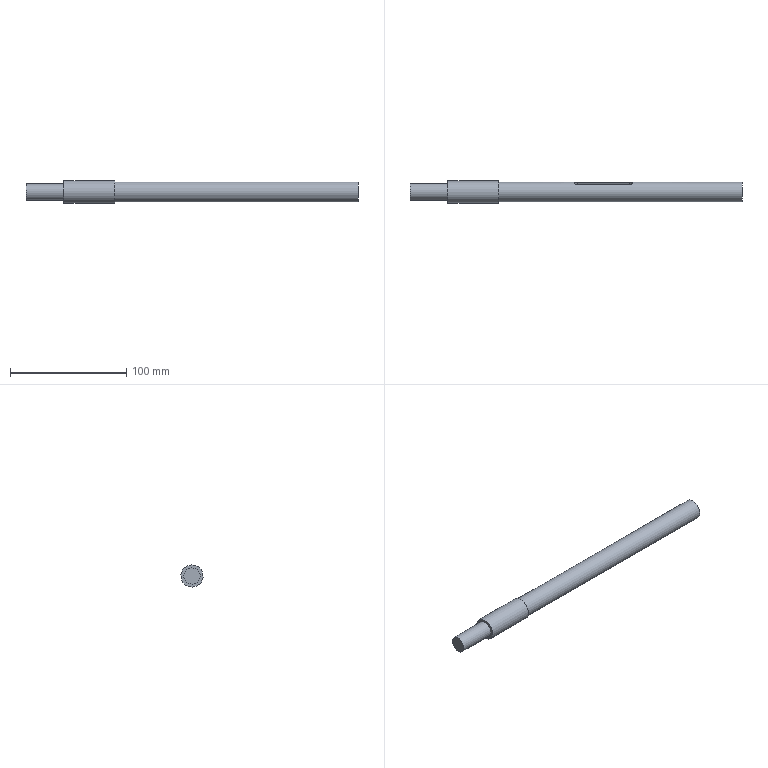Component | NX | SHAFT | 1 solid | 12 faces | box 285 x 19 x 19 mm | volume 64194 mm3 | plane 7 | cylinder 5 | commonest cylinder face diameters 5 x2 17 x1 14 x1 19 x1
STEP:
#1=CARTESIAN_POINT('',(0.,0.,0.));
#2=DIRECTION('',(0.,0.,1.));
#3=DIRECTION('',(1.,0.,0.));
#4=AXIS2_PLACEMENT_3D('',#1,#2,#3);
#5=CARTESIAN_POINT('',(190.,-3.867,130.57));
#6=VERTEX_POINT('',#5);
#7=CARTESIAN_POINT('',(190.,-0.,123.));
#8=DIRECTION('',(1.,0.,0.));
#9=DIRECTION('',(0.,-0.4549,0.8906));
#10=AXIS2_PLACEMENT_3D('',#7,#8,#9);
#11=CIRCLE('',#10,8.5);
#12=CARTESIAN_POINT('',(-19.,-0.,123.));
#13=DIRECTION('',(1.,0.,0.));
#14=DIRECTION('',(0.,-0.4549,0.8906));
#15=AXIS2_PLACEMENT_3D('',#12,#13,#14);
#16=CYLINDRICAL_SURFACE('',#15,8.5);
#17=CARTESIAN_POINT('',(0.,209.));
#18=DIRECTION('',(1.,0.));
#19=VECTOR('',#18,1.);
#20=LINE('',#17,#19);
#21=(GEOMETRIC_REPRESENTATION_CONTEXT(2)PARAMETRIC_REPRESENTATION_CONTEXT()REPRESENTATION_CONTEXT('',''));
#22=DEFINITIONAL_REPRESENTATION('',(#20),#21);
#23=PCURVE('',#16,#22);
#24=CARTESIAN_POINT('',(190.,-0.,123.));
#25=DIRECTION('',(1.,0.,0.));
#26=DIRECTION('',(0.,-0.4549,0.8906));
#27=AXIS2_PLACEMENT_3D('',#24,#25,#26);
#28=PLANE('',#27);
#29=CARTESIAN_POINT('',(0.,0.));
#30=DIRECTION('',(1.,-0.));
#31=AXIS2_PLACEMENT_2D('',#29,#30);
#32=CIRCLE('',#31,8.5);
#33=(GEOMETRIC_REPRESENTATION_CONTEXT(2)PARAMETRIC_REPRESENTATION_CONTEXT()REPRESENTATION_CONTEXT('',''));
#34=DEFINITIONAL_REPRESENTATION('',(#32),#33);
#35=PCURVE('',#28,#34);
#36=SURFACE_CURVE('',#11,(#23,#35),.PCURVE_S1.);
#37=EDGE_CURVE('',#6,#6,#36,.T.);
#38=ORIENTED_EDGE('',*,*,#37,.F.);
#39=CARTESIAN_POINT('',(-19.,-3.867,130.57));
#40=VERTEX_POINT('',#39);
#41=CARTESIAN_POINT('',(-19.,-3.867,130.57));
#42=CARTESIAN_POINT('',(190.,-3.867,130.57));
#43=B_SPLINE_CURVE_WITH_KNOTS('',1,(#41,#42),.UNSPECIFIED.,.F.,.F.,(2,2),(0.,209.),.PIECEWISE_BEZIER_KNOTS.);
#44=CARTESIAN_POINT('',(0.,0.));
#45=DIRECTION('',(0.,1.));
#46=VECTOR('',#45,1.);
#47=LINE('',#44,#46);
#48=(GEOMETRIC_REPRESENTATION_CONTEXT(2)PARAMETRIC_REPRESENTATION_CONTEXT()REPRESENTATION_CONTEXT('',''));
#49=DEFINITIONAL_REPRESENTATION('',(#47),#48);
#50=PCURVE('',#16,#49);
#51=CARTESIAN_POINT('',(6.283,0.));
#52=DIRECTION('',(0.,1.));
#53=VECTOR('',#52,1.);
#54=LINE('',#51,#53);
#55=(GEOMETRIC_REPRESENTATION_CONTEXT(2)PARAMETRIC_REPRESENTATION_CONTEXT()REPRESENTATION_CONTEXT('',''));
#56=DEFINITIONAL_REPRESENTATION('',(#54),#55);
#57=PCURVE('',#16,#56);
#58=SEAM_CURVE('',#43,(#50,#57),.PCURVE_S1.);
#59=EDGE_CURVE('',#40,#6,#58,.T.);
#60=ORIENTED_EDGE('',*,*,#59,.F.);
#61=CARTESIAN_POINT('',(-19.,-0.,123.));
#62=DIRECTION('',(1.,0.,0.));
#63=DIRECTION('',(0.,-0.4549,0.8906));
#64=AXIS2_PLACEMENT_3D('',#61,#62,#63);
#65=CIRCLE('',#64,8.5);
#66=CARTESIAN_POINT('',(0.,0.));
#67=DIRECTION('',(1.,0.));
#68=VECTOR('',#67,1.);
#69=LINE('',#66,#68);
#70=(GEOMETRIC_REPRESENTATION_CONTEXT(2)PARAMETRIC_REPRESENTATION_CONTEXT()REPRESENTATION_CONTEXT('',''));
#71=DEFINITIONAL_REPRESENTATION('',(#69),#70);
#72=PCURVE('',#16,#71);
#73=CARTESIAN_POINT('',(-19.,-0.,123.));
#74=DIRECTION('',(1.,0.,0.));
#75=DIRECTION('',(0.,-0.4549,0.8906));
#76=AXIS2_PLACEMENT_3D('',#73,#74,#75);
#77=PLANE('',#76);
#78=CARTESIAN_POINT('',(-0.,-0.));
#79=DIRECTION('',(1.,-0.));
#80=AXIS2_PLACEMENT_2D('',#78,#79);
#81=CIRCLE('',#80,8.5);
#82=(GEOMETRIC_REPRESENTATION_CONTEXT(2)PARAMETRIC_REPRESENTATION_CONTEXT()REPRESENTATION_CONTEXT('',''));
#83=DEFINITIONAL_REPRESENTATION('',(#81),#82);
#84=PCURVE('',#77,#83);
#85=SURFACE_CURVE('',#65,(#72,#84),.PCURVE_S1.);
#86=EDGE_CURVE('',#40,#40,#85,.T.);
#87=ORIENTED_EDGE('',*,*,#86,.T.);
#88=ORIENTED_EDGE('',*,*,#59,.T.);
#89=EDGE_LOOP('',(#38,#60,#87,#88));
#90=FACE_BOUND('',#89,.T.);
#91=CARTESIAN_POINT('',(48.5,6.098,128.922));
#92=VERTEX_POINT('',#91);
#93=CARTESIAN_POINT('',(48.5,8.372,124.469));
#94=VERTEX_POINT('',#93);
#95=CARTESIAN_POINT('',(48.5,6.098,128.922));
#96=CARTESIAN_POINT('',(48.227,6.098,128.922));
#97=CARTESIAN_POINT('',(47.95,6.132,128.887));
#98=CARTESIAN_POINT('',(47.693,6.194,128.821));
#99=CARTESIAN_POINT('',(47.436,6.257,128.754));
#100=CARTESIAN_POINT('',(47.191,6.349,128.654));
#101=CARTESIAN_POINT('',(46.977,6.459,128.526));
#102=CARTESIAN_POINT('',(46.757,6.572,128.394));
#103=CARTESIAN_POINT('',(46.564,6.706,128.228));
#104=CARTESIAN_POINT('',(46.411,6.845,128.039));
#105=CARTESIAN_POINT('',(46.256,6.987,127.846));
#106=CARTESIAN_POINT('',(46.139,7.139,127.622));
#107=CARTESIAN_POINT('',(46.071,7.282,127.385));
#108=CARTESIAN_POINT('',(46.006,7.421,127.153));
#109=CARTESIAN_POINT('',(45.985,7.556,126.902));
#110=CARTESIAN_POINT('',(46.011,7.675,126.653));
#111=CARTESIAN_POINT('',(46.037,7.79,126.411));
#112=CARTESIAN_POINT('',(46.108,7.893,126.163));
#113=CARTESIAN_POINT('',(46.217,7.978,125.932));
#114=CARTESIAN_POINT('',(46.327,8.064,125.698));
#115=CARTESIAN_POINT('',(46.479,8.134,125.475));
#116=CARTESIAN_POINT('',(46.662,8.189,125.28));
#117=CARTESIAN_POINT('',(46.851,8.245,125.078));
#118=CARTESIAN_POINT('',(47.078,8.286,124.902));
#119=CARTESIAN_POINT('',(47.326,8.314,124.768));
#120=CARTESIAN_POINT('',(47.575,8.343,124.634));
#121=CARTESIAN_POINT('',(47.853,8.36,124.54));
#122=CARTESIAN_POINT('',(48.135,8.367,124.497));
#123=CARTESIAN_POINT('',(48.255,8.37,124.478));
#124=CARTESIAN_POINT('',(48.378,8.372,124.469));
#125=CARTESIAN_POINT('',(48.5,8.372,124.469));
#126=B_SPLINE_CURVE_WITH_KNOTS('',3,(#95,#96,#97,#98,#99,#100,#101,#102,#103,#104,#105,#106,#107,#108,#109,#110,#111,#112,#113,#114,#115,#116,#117,#118,#119,#120,#121,#122,#123,#124,#125),.UNSPECIFIED.,.F.,.F.,(4,3,3,3,3,3,3,3,3,3,4),(0.,0.1042,0.2083,0.3152,0.4244,0.5305,0.6332,0.7372,0.845,0.9539,1.),.UNSPECIFIED.);
#127=CARTESIAN_POINT('',(5.011,67.5));
#128=CARTESIAN_POINT('',(5.011,67.44));
#129=CARTESIAN_POINT('',(5.01,67.321));
#130=CARTESIAN_POINT('',(5.008,67.142));
#131=CARTESIAN_POINT('',(5.004,66.965));
#132=CARTESIAN_POINT('',(4.999,66.792));
#133=CARTESIAN_POINT('',(4.992,66.623));
#134=CARTESIAN_POINT('',(4.983,66.458));
#135=CARTESIAN_POINT('',(4.974,66.298));
#136=CARTESIAN_POINT('',(4.962,66.145));
#137=CARTESIAN_POINT('',(4.95,65.999));
#138=CARTESIAN_POINT('',(4.937,65.862));
#139=CARTESIAN_POINT('',(4.922,65.731));
#140=CARTESIAN_POINT('',(4.906,65.61));
#141=CARTESIAN_POINT('',(4.89,65.498));
#142=CARTESIAN_POINT('',(4.873,65.397));
#143=CARTESIAN_POINT('',(4.854,65.306));
#144=CARTESIAN_POINT('',(4.835,65.226));
#145=CARTESIAN_POINT('',(4.816,65.157));
#146=CARTESIAN_POINT('',(4.796,65.1));
#147=CARTESIAN_POINT('',(4.776,65.056));
#148=CARTESIAN_POINT('',(4.755,65.024));
#149=CARTESIAN_POINT('',(4.734,65.005));
#150=CARTESIAN_POINT('',(4.713,64.998));
#151=CARTESIAN_POINT('',(4.691,65.004));
#152=CARTESIAN_POINT('',(4.671,65.023));
#153=CARTESIAN_POINT('',(4.65,65.055));
#154=CARTESIAN_POINT('',(4.629,65.1));
#155=CARTESIAN_POINT('',(4.609,65.157));
#156=CARTESIAN_POINT('',(4.59,65.225));
#157=CARTESIAN_POINT('',(4.571,65.305));
#158=CARTESIAN_POINT('',(4.552,65.396));
#159=CARTESIAN_POINT('',(4.535,65.498));
#160=CARTESIAN_POINT('',(4.518,65.609));
#161=CARTESIAN_POINT('',(4.503,65.729));
#162=CARTESIAN_POINT('',(4.488,65.859));
#163=CARTESIAN_POINT('',(4.475,65.998));
#164=CARTESIAN_POINT('',(4.462,66.144));
#165=CARTESIAN_POINT('',(4.451,66.297));
#166=CARTESIAN_POINT('',(4.442,66.455));
#167=CARTESIAN_POINT('',(4.433,66.62));
#168=CARTESIAN_POINT('',(4.426,66.79));
#169=CARTESIAN_POINT('',(4.421,66.964));
#170=CARTESIAN_POINT('',(4.417,67.139));
#171=CARTESIAN_POINT('',(4.414,67.319));
#172=CARTESIAN_POINT('',(4.414,67.44));
#173=CARTESIAN_POINT('',(4.414,67.5));
#174=B_SPLINE_CURVE_WITH_KNOTS('',3,(#127,#128,#129,#130,#131,#132,#133,#134,#135,#136,#137,#138,#139,#140,#141,#142,#143,#144,#145,#146,#147,#148,#149,#150,#151,#152,#153,#154,#155,#156,#157,#158,#159,#160,#161,#162,#163,#164,#165,#166,#167,#168,#169,#170,#171,#172,#173),.UNSPECIFIED.,.F.,.F.,(4,1,1,1,1,1,1,1,1,1,1,1,1,1,1,1,1,1,1,1,1,1,1,1,1,1,1,1,1,1,1,1,1,1,1,1,1,1,1,1,1,1,1,1,4),(0.,0.02273,0.04545,0.06818,0.09091,0.1136,0.1364,0.1591,0.1818,0.2045,0.2273,0.25,0.2727,0.2955,0.3182,0.3409,0.3636,0.3864,0.4091,0.4318,0.4545,0.4773,0.5,0.5227,0.5455,0.5682,0.5909,0.6136,0.6364,0.6591,0.6818,0.7045,0.7273,0.75,0.7727,0.7955,0.8182,0.8409,0.8636,0.8864,0.9091,0.9318,0.9545,0.9773,1.),.QUASI_UNIFORM_KNOTS.);
#175=(GEOMETRIC_REPRESENTATION_CONTEXT(2)PARAMETRIC_REPRESENTATION_CONTEXT()REPRESENTATION_CONTEXT('',''));
#176=DEFINITIONAL_REPRESENTATION('',(#174),#175);
#177=PCURVE('',#16,#176);
#178=CARTESIAN_POINT('',(48.5,44.528,145.744));
#179=DIRECTION('',(0.,-0.8906,-0.4549));
#180=DIRECTION('',(1.,0.,0.));
#181=AXIS2_PLACEMENT_3D('',#178,#179,#180);
#182=CYLINDRICAL_SURFACE('',#181,2.5);
#183=CARTESIAN_POINT('',(1.571,41.876));
#184=CARTESIAN_POINT('',(1.595,41.876));
#185=CARTESIAN_POINT('',(1.642,41.875));
#186=CARTESIAN_POINT('',(1.714,41.869));
#187=CARTESIAN_POINT('',(1.786,41.859));
#188=CARTESIAN_POINT('',(1.858,41.846));
#189=CARTESIAN_POINT('',(1.929,41.829));
#190=CARTESIAN_POINT('',(2.,41.81));
#191=CARTESIAN_POINT('',(2.072,41.788));
#192=CARTESIAN_POINT('',(2.143,41.764));
#193=CARTESIAN_POINT('',(2.214,41.739));
#194=CARTESIAN_POINT('',(2.285,41.713));
#195=CARTESIAN_POINT('',(2.356,41.686));
#196=CARTESIAN_POINT('',(2.427,41.659));
#197=CARTESIAN_POINT('',(2.498,41.633));
#198=CARTESIAN_POINT('',(2.569,41.608));
#199=CARTESIAN_POINT('',(2.64,41.585));
#200=CARTESIAN_POINT('',(2.711,41.564));
#201=CARTESIAN_POINT('',(2.783,41.545));
#202=CARTESIAN_POINT('',(2.854,41.529));
#203=CARTESIAN_POINT('',(2.926,41.516));
#204=CARTESIAN_POINT('',(2.997,41.507));
#205=CARTESIAN_POINT('',(3.069,41.501));
#206=CARTESIAN_POINT('',(3.141,41.499));
#207=CARTESIAN_POINT('',(3.213,41.501));
#208=CARTESIAN_POINT('',(3.284,41.507));
#209=CARTESIAN_POINT('',(3.356,41.516));
#210=CARTESIAN_POINT('',(3.428,41.529));
#211=CARTESIAN_POINT('',(3.5,41.545));
#212=CARTESIAN_POINT('',(3.571,41.563));
#213=CARTESIAN_POINT('',(3.642,41.585));
#214=CARTESIAN_POINT('',(3.713,41.608));
#215=CARTESIAN_POINT('',(3.784,41.633));
#216=CARTESIAN_POINT('',(3.856,41.659));
#217=CARTESIAN_POINT('',(3.926,41.686));
#218=CARTESIAN_POINT('',(3.997,41.712));
#219=CARTESIAN_POINT('',(4.068,41.739));
#220=CARTESIAN_POINT('',(4.14,41.764));
#221=CARTESIAN_POINT('',(4.211,41.788));
#222=CARTESIAN_POINT('',(4.282,41.81));
#223=CARTESIAN_POINT('',(4.353,41.829));
#224=CARTESIAN_POINT('',(4.425,41.845));
#225=CARTESIAN_POINT('',(4.496,41.859));
#226=CARTESIAN_POINT('',(4.567,41.869));
#227=CARTESIAN_POINT('',(4.64,41.875));
#228=CARTESIAN_POINT('',(4.688,41.876));
#229=CARTESIAN_POINT('',(4.712,41.876));
#230=B_SPLINE_CURVE_WITH_KNOTS('',3,(#183,#184,#185,#186,#187,#188,#189,#190,#191,#192,#193,#194,#195,#196,#197,#198,#199,#200,#201,#202,#203,#204,#205,#206,#207,#208,#209,#210,#211,#212,#213,#214,#215,#216,#217,#218,#219,#220,#221,#222,#223,#224,#225,#226,#227,#228,#229),.UNSPECIFIED.,.F.,.F.,(4,1,1,1,1,1,1,1,1,1,1,1,1,1,1,1,1,1,1,1,1,1,1,1,1,1,1,1,1,1,1,1,1,1,1,1,1,1,1,1,1,1,1,1,4),(0.,0.02273,0.04545,0.06818,0.09091,0.1136,0.1364,0.1591,0.1818,0.2045,0.2273,0.25,0.2727,0.2955,0.3182,0.3409,0.3636,0.3864,0.4091,0.4318,0.4545,0.4773,0.5,0.5227,0.5455,0.5682,0.5909,0.6136,0.6364,0.6591,0.6818,0.7045,0.7273,0.75,0.7727,0.7955,0.8182,0.8409,0.8636,0.8864,0.9091,0.9318,0.9545,0.9773,1.),.QUASI_UNIFORM_KNOTS.);
#231=(GEOMETRIC_REPRESENTATION_CONTEXT(2)PARAMETRIC_REPRESENTATION_CONTEXT()REPRESENTATION_CONTEXT('',''));
#232=DEFINITIONAL_REPRESENTATION('',(#230),#231);
#233=PCURVE('',#182,#232);
#234=SURFACE_CURVE('',#126,(#177,#233),.PCURVE_S1.);
#235=EDGE_CURVE('',#92,#94,#234,.T.);
#236=ORIENTED_EDGE('',*,*,#235,.T.);
#237=CARTESIAN_POINT('',(93.5,8.372,124.469));
#238=VERTEX_POINT('',#237);
#239=CARTESIAN_POINT('',(-19.,8.372,124.469));
#240=DIRECTION('',(1.,0.,0.));
#241=VECTOR('',#240,1.);
#242=LINE('',#239,#241);
#243=CARTESIAN_POINT('',(4.414,0.));
#244=DIRECTION('',(0.,1.));
#245=VECTOR('',#244,1.);
#246=LINE('',#243,#245);
#247=(GEOMETRIC_REPRESENTATION_CONTEXT(2)PARAMETRIC_REPRESENTATION_CONTEXT()REPRESENTATION_CONTEXT('',''));
#248=DEFINITIONAL_REPRESENTATION('',(#246),#247);
#249=PCURVE('',#16,#248);
#250=CARTESIAN_POINT('',(93.5,45.665,143.518));
#251=DIRECTION('',(-0.,-0.4549,0.8906));
#252=DIRECTION('',(-1.,0.,-0.));
#253=AXIS2_PLACEMENT_3D('',#250,#251,#252);
#254=PLANE('',#253);
#255=CARTESIAN_POINT('',(112.5,41.876));
#256=DIRECTION('',(-1.,-0.));
#257=VECTOR('',#256,1.);
#258=LINE('',#255,#257);
#259=(GEOMETRIC_REPRESENTATION_CONTEXT(2)PARAMETRIC_REPRESENTATION_CONTEXT()REPRESENTATION_CONTEXT('',''));
#260=DEFINITIONAL_REPRESENTATION('',(#258),#259);
#261=PCURVE('',#254,#260);
#262=SURFACE_CURVE('',#242,(#249,#261),.PCURVE_S1.);
#263=EDGE_CURVE('',#94,#238,#262,.T.);
#264=ORIENTED_EDGE('',*,*,#263,.T.);
#265=CARTESIAN_POINT('',(93.5,6.098,128.922));
#266=VERTEX_POINT('',#265);
#267=CARTESIAN_POINT('',(93.5,8.372,124.469));
#268=CARTESIAN_POINT('',(93.773,8.372,124.469));
#269=CARTESIAN_POINT('',(94.05,8.364,124.517));
#270=CARTESIAN_POINT('',(94.307,8.347,124.606));
#271=CARTESIAN_POINT('',(94.564,8.33,124.696));
#272=CARTESIAN_POINT('',(94.809,8.302,124.83));
#273=CARTESIAN_POINT('',(95.023,8.263,124.994));
#274=CARTESIAN_POINT('',(95.243,8.222,125.163));
#275=CARTESIAN_POINT('',(95.436,8.167,125.368));
#276=CARTESIAN_POINT('',(95.589,8.095,125.592));
#277=CARTESIAN_POINT('',(95.744,8.022,125.821));
#278=CARTESIAN_POINT('',(95.861,7.929,126.074));
#279=CARTESIAN_POINT('',(95.929,7.821,126.33));
#280=CARTESIAN_POINT('',(95.994,7.715,126.578));
#281=CARTESIAN_POINT('',(96.015,7.591,126.835));
#282=CARTESIAN_POINT('',(95.989,7.458,127.077));
#283=CARTESIAN_POINT('',(95.963,7.33,127.313));
#284=CARTESIAN_POINT('',(95.892,7.19,127.541));
#285=CARTESIAN_POINT('',(95.783,7.052,127.745));
#286=CARTESIAN_POINT('',(95.673,6.913,127.952));
#287=CARTESIAN_POINT('',(95.521,6.773,128.14));
#288=CARTESIAN_POINT('',(95.338,6.647,128.298));
#289=CARTESIAN_POINT('',(95.149,6.516,128.462));
#290=CARTESIAN_POINT('',(94.922,6.397,128.598));
#291=CARTESIAN_POINT('',(94.674,6.306,128.699));
#292=CARTESIAN_POINT('',(94.425,6.214,128.801));
#293=CARTESIAN_POINT('',(94.147,6.147,128.87));
#294=CARTESIAN_POINT('',(93.865,6.117,128.902));
#295=CARTESIAN_POINT('',(93.745,6.104,128.915));
#296=CARTESIAN_POINT('',(93.622,6.098,128.922));
#297=CARTESIAN_POINT('',(93.5,6.098,128.922));
#298=B_SPLINE_CURVE_WITH_KNOTS('',3,(#267,#268,#269,#270,#271,#272,#273,#274,#275,#276,#277,#278,#279,#280,#281,#282,#283,#284,#285,#286,#287,#288,#289,#290,#291,#292,#293,#294,#295,#296,#297),.UNSPECIFIED.,.F.,.F.,(4,3,3,3,3,3,3,3,3,3,4),(0.,0.1042,0.2083,0.3152,0.4244,0.5305,0.6332,0.7372,0.845,0.9539,1.),.UNSPECIFIED.);
#299=CARTESIAN_POINT('',(4.414,112.5));
#300=CARTESIAN_POINT('',(4.414,112.56));
#301=CARTESIAN_POINT('',(4.414,112.679));
#302=CARTESIAN_POINT('',(4.417,112.858));
#303=CARTESIAN_POINT('',(4.421,113.035));
#304=CARTESIAN_POINT('',(4.426,113.208));
#305=CARTESIAN_POINT('',(4.433,113.377));
#306=CARTESIAN_POINT('',(4.441,113.542));
#307=CARTESIAN_POINT('',(4.451,113.702));
#308=CARTESIAN_POINT('',(4.462,113.855));
#309=CARTESIAN_POINT('',(4.475,114.001));
#310=CARTESIAN_POINT('',(4.488,114.138));
#311=CARTESIAN_POINT('',(4.503,114.269));
#312=CARTESIAN_POINT('',(4.518,114.39));
#313=CARTESIAN_POINT('',(4.535,114.502));
#314=CARTESIAN_POINT('',(4.552,114.603));
#315=CARTESIAN_POINT('',(4.57,114.694));
#316=CARTESIAN_POINT('',(4.589,114.774));
#317=CARTESIAN_POINT('',(4.609,114.843));
#318=CARTESIAN_POINT('',(4.629,114.9));
#319=CARTESIAN_POINT('',(4.649,114.944));
#320=CARTESIAN_POINT('',(4.67,114.976));
#321=CARTESIAN_POINT('',(4.691,114.995));
#322=CARTESIAN_POINT('',(4.712,115.002));
#323=CARTESIAN_POINT('',(4.733,114.996));
#324=CARTESIAN_POINT('',(4.754,114.977));
#325=CARTESIAN_POINT('',(4.775,114.945));
#326=CARTESIAN_POINT('',(4.796,114.9));
#327=CARTESIAN_POINT('',(4.816,114.843));
#328=CARTESIAN_POINT('',(4.835,114.775));
#329=CARTESIAN_POINT('',(4.854,114.695));
#330=CARTESIAN_POINT('',(4.872,114.604));
#331=CARTESIAN_POINT('',(4.89,114.502));
#332=CARTESIAN_POINT('',(4.906,114.391));
#333=CARTESIAN_POINT('',(4.922,114.271));
#334=CARTESIAN_POINT('',(4.936,114.141));
#335=CARTESIAN_POINT('',(4.95,114.002));
#336=CARTESIAN_POINT('',(4.962,113.856));
#337=CARTESIAN_POINT('',(4.973,113.703));
#338=CARTESIAN_POINT('',(4.983,113.545));
#339=CARTESIAN_POINT('',(4.992,113.38));
#340=CARTESIAN_POINT('',(4.999,113.21));
#341=CARTESIAN_POINT('',(5.004,113.036));
#342=CARTESIAN_POINT('',(5.008,112.861));
#343=CARTESIAN_POINT('',(5.01,112.681));
#344=CARTESIAN_POINT('',(5.011,112.56));
#345=CARTESIAN_POINT('',(5.011,112.5));
#346=B_SPLINE_CURVE_WITH_KNOTS('',3,(#299,#300,#301,#302,#303,#304,#305,#306,#307,#308,#309,#310,#311,#312,#313,#314,#315,#316,#317,#318,#319,#320,#321,#322,#323,#324,#325,#326,#327,#328,#329,#330,#331,#332,#333,#334,#335,#336,#337,#338,#339,#340,#341,#342,#343,#344,#345),.UNSPECIFIED.,.F.,.F.,(4,1,1,1,1,1,1,1,1,1,1,1,1,1,1,1,1,1,1,1,1,1,1,1,1,1,1,1,1,1,1,1,1,1,1,1,1,1,1,1,1,1,1,1,4),(0.,0.02273,0.04545,0.06818,0.09091,0.1136,0.1364,0.1591,0.1818,0.2045,0.2273,0.25,0.2727,0.2955,0.3182,0.3409,0.3636,0.3864,0.4091,0.4318,0.4545,0.4773,0.5,0.5227,0.5455,0.5682,0.5909,0.6136,0.6364,0.6591,0.6818,0.7045,0.7273,0.75,0.7727,0.7955,0.8182,0.8409,0.8636,0.8864,0.9091,0.9318,0.9545,0.9773,1.),.QUASI_UNIFORM_KNOTS.);
#347=(GEOMETRIC_REPRESENTATION_CONTEXT(2)PARAMETRIC_REPRESENTATION_CONTEXT()REPRESENTATION_CONTEXT('',''));
#348=DEFINITIONAL_REPRESENTATION('',(#346),#347);
#349=PCURVE('',#16,#348);
#350=CARTESIAN_POINT('',(93.5,44.528,145.744));
#351=DIRECTION('',(0.,-0.8906,-0.4549));
#352=DIRECTION('',(1.,0.,0.));
#353=AXIS2_PLACEMENT_3D('',#350,#351,#352);
#354=CYLINDRICAL_SURFACE('',#353,2.5);
#355=CARTESIAN_POINT('',(4.712,41.876));
#356=CARTESIAN_POINT('',(4.736,41.876));
#357=CARTESIAN_POINT('',(4.784,41.875));
#358=CARTESIAN_POINT('',(4.856,41.869));
#359=CARTESIAN_POINT('',(4.928,41.859));
#360=CARTESIAN_POINT('',(4.999,41.846));
#361=CARTESIAN_POINT('',(5.07,41.829));
#362=CARTESIAN_POINT('',(5.142,41.81));
#363=CARTESIAN_POINT('',(5.213,41.788));
#364=CARTESIAN_POINT('',(5.285,41.764));
#365=CARTESIAN_POINT('',(5.356,41.739));
#366=CARTESIAN_POINT('',(5.426,41.713));
#367=CARTESIAN_POINT('',(5.497,41.686));
#368=CARTESIAN_POINT('',(5.569,41.659));
#369=CARTESIAN_POINT('',(5.64,41.633));
#370=CARTESIAN_POINT('',(5.711,41.608));
#371=CARTESIAN_POINT('',(5.782,41.585));
#372=CARTESIAN_POINT('',(5.853,41.564));
#373=CARTESIAN_POINT('',(5.925,41.545));
#374=CARTESIAN_POINT('',(5.996,41.529));
#375=CARTESIAN_POINT('',(6.067,41.516));
#376=CARTESIAN_POINT('',(6.139,41.507));
#377=CARTESIAN_POINT('',(6.211,41.501));
#378=CARTESIAN_POINT('',(6.283,41.499));
#379=CARTESIAN_POINT('',(6.354,41.501));
#380=CARTESIAN_POINT('',(6.426,41.507));
#381=CARTESIAN_POINT('',(6.498,41.516));
#382=CARTESIAN_POINT('',(6.569,41.529));
#383=CARTESIAN_POINT('',(6.641,41.545));
#384=CARTESIAN_POINT('',(6.712,41.563));
#385=CARTESIAN_POINT('',(6.783,41.585));
#386=CARTESIAN_POINT('',(6.855,41.608));
#387=CARTESIAN_POINT('',(6.926,41.633));
#388=CARTESIAN_POINT('',(6.997,41.659));
#389=CARTESIAN_POINT('',(7.068,41.686));
#390=CARTESIAN_POINT('',(7.139,41.712));
#391=CARTESIAN_POINT('',(7.21,41.739));
#392=CARTESIAN_POINT('',(7.281,41.764));
#393=CARTESIAN_POINT('',(7.352,41.788));
#394=CARTESIAN_POINT('',(7.423,41.81));
#395=CARTESIAN_POINT('',(7.495,41.829));
#396=CARTESIAN_POINT('',(7.566,41.845));
#397=CARTESIAN_POINT('',(7.638,41.859));
#398=CARTESIAN_POINT('',(7.709,41.869));
#399=CARTESIAN_POINT('',(7.782,41.875));
#400=CARTESIAN_POINT('',(7.83,41.876));
#401=CARTESIAN_POINT('',(7.854,41.876));
#402=B_SPLINE_CURVE_WITH_KNOTS('',3,(#355,#356,#357,#358,#359,#360,#361,#362,#363,#364,#365,#366,#367,#368,#369,#370,#371,#372,#373,#374,#375,#376,#377,#378,#379,#380,#381,#382,#383,#384,#385,#386,#387,#388,#389,#390,#391,#392,#393,#394,#395,#396,#397,#398,#399,#400,#401),.UNSPECIFIED.,.F.,.F.,(4,1,1,1,1,1,1,1,1,1,1,1,1,1,1,1,1,1,1,1,1,1,1,1,1,1,1,1,1,1,1,1,1,1,1,1,1,1,1,1,1,1,1,1,4),(0.,0.02273,0.04545,0.06818,0.09091,0.1136,0.1364,0.1591,0.1818,0.2045,0.2273,0.25,0.2727,0.2955,0.3182,0.3409,0.3636,0.3864,0.4091,0.4318,0.4545,0.4773,0.5,0.5227,0.5455,0.5682,0.5909,0.6136,0.6364,0.6591,0.6818,0.7045,0.7273,0.75,0.7727,0.7955,0.8182,0.8409,0.8636,0.8864,0.9091,0.9318,0.9545,0.9773,1.),.QUASI_UNIFORM_KNOTS.);
#403=(GEOMETRIC_REPRESENTATION_CONTEXT(2)PARAMETRIC_REPRESENTATION_CONTEXT()REPRESENTATION_CONTEXT('',''));
#404=DEFINITIONAL_REPRESENTATION('',(#402),#403);
#405=PCURVE('',#354,#404);
#406=SURFACE_CURVE('',#298,(#349,#405),.PCURVE_S1.);
#407=EDGE_CURVE('',#238,#266,#406,.T.);
#408=ORIENTED_EDGE('',*,*,#407,.T.);
#409=CARTESIAN_POINT('',(-19.,6.098,128.922));
#410=DIRECTION('',(-1.,0.,0.));
#411=VECTOR('',#410,1.);
#412=LINE('',#409,#411);
#413=CARTESIAN_POINT('',(5.011,0.));
#414=DIRECTION('',(0.,-1.));
#415=VECTOR('',#414,1.);
#416=LINE('',#413,#415);
#417=(GEOMETRIC_REPRESENTATION_CONTEXT(2)PARAMETRIC_REPRESENTATION_CONTEXT()REPRESENTATION_CONTEXT('',''));
#418=DEFINITIONAL_REPRESENTATION('',(#416),#417);
#419=PCURVE('',#16,#418);
#420=CARTESIAN_POINT('',(48.5,43.39,147.971));
#421=DIRECTION('',(-0.,0.4549,-0.8906));
#422=DIRECTION('',(1.,0.,-0.));
#423=AXIS2_PLACEMENT_3D('',#420,#421,#422);
#424=PLANE('',#423);
#425=CARTESIAN_POINT('',(-67.5,41.876));
#426=DIRECTION('',(-1.,-0.));
#427=VECTOR('',#426,1.);
#428=LINE('',#425,#427);
#429=(GEOMETRIC_REPRESENTATION_CONTEXT(2)PARAMETRIC_REPRESENTATION_CONTEXT()REPRESENTATION_CONTEXT('',''));
#430=DEFINITIONAL_REPRESENTATION('',(#428),#429);
#431=PCURVE('',#424,#430);
#432=SURFACE_CURVE('',#412,(#419,#431),.PCURVE_S1.);
#433=EDGE_CURVE('',#266,#92,#432,.T.);
#434=ORIENTED_EDGE('',*,*,#433,.T.);
#435=EDGE_LOOP('',(#236,#264,#408,#434));
#436=FACE_BOUND('',#435,.T.);
#437=ADVANCED_FACE('',(#90,#436),#16,.T.);
#438=CARTESIAN_POINT('',(-95.,-3.184,129.234));
#439=VERTEX_POINT('',#438);
#440=CARTESIAN_POINT('',(-95.,-0.,123.));
#441=DIRECTION('',(1.,0.,0.));
#442=DIRECTION('',(0.,-0.4549,0.8906));
#443=AXIS2_PLACEMENT_3D('',#440,#441,#442);
#444=CIRCLE('',#443,7.);
#445=CARTESIAN_POINT('',(-95.,-0.,123.));
#446=DIRECTION('',(-1.,0.,0.));
#447=DIRECTION('',(0.,0.4549,-0.8906));
#448=AXIS2_PLACEMENT_3D('',#445,#446,#447);
#449=PLANE('',#448);
#450=CARTESIAN_POINT('',(-7.,0.));
#451=CARTESIAN_POINT('',(-7.,12.124));
#452=CARTESIAN_POINT('',(3.5,6.062));
#453=CARTESIAN_POINT('',(14.,0.));
#454=CARTESIAN_POINT('',(3.5,-6.062));
#455=CARTESIAN_POINT('',(-7.,-12.124));
#456=CARTESIAN_POINT('',(-7.,0.));
#457=(BOUNDED_CURVE()B_SPLINE_CURVE(2,(#450,#451,#452,#453,#454,#455,#456),.UNSPECIFIED.,.T.,.F.)B_SPLINE_CURVE_WITH_KNOTS((1,2,2,2,2,1),(-2.094,0.,2.094,4.189,6.283,8.378),.UNSPECIFIED.)CURVE()GEOMETRIC_REPRESENTATION_ITEM()RATIONAL_B_SPLINE_CURVE((1.,0.5,1.,0.5,1.,0.5,1.))REPRESENTATION_ITEM(''));
#458=(GEOMETRIC_REPRESENTATION_CONTEXT(2)PARAMETRIC_REPRESENTATION_CONTEXT()REPRESENTATION_CONTEXT('',''));
#459=DEFINITIONAL_REPRESENTATION('',(#457),#458);
#460=PCURVE('',#449,#459);
#461=CARTESIAN_POINT('',(-95.,-0.,123.));
#462=DIRECTION('',(1.,0.,0.));
#463=DIRECTION('',(0.,-0.4549,0.8906));
#464=AXIS2_PLACEMENT_3D('',#461,#462,#463);
#465=CYLINDRICAL_SURFACE('',#464,7.);
#466=CARTESIAN_POINT('',(0.,0.));
#467=DIRECTION('',(1.,0.));
#468=VECTOR('',#467,1.);
#469=LINE('',#466,#468);
#470=(GEOMETRIC_REPRESENTATION_CONTEXT(2)PARAMETRIC_REPRESENTATION_CONTEXT()REPRESENTATION_CONTEXT('',''));
#471=DEFINITIONAL_REPRESENTATION('',(#469),#470);
#472=PCURVE('',#465,#471);
#473=SURFACE_CURVE('',#444,(#460,#472),.PCURVE_S1.);
#474=EDGE_CURVE('',#439,#439,#473,.T.);
#475=ORIENTED_EDGE('',*,*,#474,.F.);
#476=EDGE_LOOP('',(#475));
#477=FACE_BOUND('',#476,.T.);
#478=ADVANCED_FACE('',(#477),#449,.T.);
#479=CARTESIAN_POINT('',(-62.5,-3.184,129.234));
#480=VERTEX_POINT('',#479);
#481=CARTESIAN_POINT('',(-62.5,-0.,123.));
#482=DIRECTION('',(-1.,0.,0.));
#483=DIRECTION('',(0.,-0.4549,0.8906));
#484=AXIS2_PLACEMENT_3D('',#481,#482,#483);
#485=CIRCLE('',#484,7.);
#486=CARTESIAN_POINT('',(6.283,32.5));
#487=DIRECTION('',(-1.,0.));
#488=VECTOR('',#487,1.);
#489=LINE('',#486,#488);
#490=(GEOMETRIC_REPRESENTATION_CONTEXT(2)PARAMETRIC_REPRESENTATION_CONTEXT()REPRESENTATION_CONTEXT('',''));
#491=DEFINITIONAL_REPRESENTATION('',(#489),#490);
#492=PCURVE('',#465,#491);
#493=CARTESIAN_POINT('',(-62.5,-0.,123.));
#494=DIRECTION('',(-1.,0.,0.));
#495=DIRECTION('',(0.,0.4549,-0.8906));
#496=AXIS2_PLACEMENT_3D('',#493,#494,#495);
#497=PLANE('',#496);
#498=CARTESIAN_POINT('',(0.,-0.));
#499=DIRECTION('',(-1.,0.));
#500=AXIS2_PLACEMENT_2D('',#498,#499);
#501=CIRCLE('',#500,7.);
#502=(GEOMETRIC_REPRESENTATION_CONTEXT(2)PARAMETRIC_REPRESENTATION_CONTEXT()REPRESENTATION_CONTEXT('',''));
#503=DEFINITIONAL_REPRESENTATION('',(#501),#502);
#504=PCURVE('',#497,#503);
#505=SURFACE_CURVE('',#485,(#492,#504),.PCURVE_S1.);
#506=EDGE_CURVE('',#480,#480,#505,.T.);
#507=ORIENTED_EDGE('',*,*,#506,.T.);
#508=CARTESIAN_POINT('',(-95.,-3.184,129.234));
#509=CARTESIAN_POINT('',(-62.5,-3.184,129.234));
#510=B_SPLINE_CURVE_WITH_KNOTS('',1,(#508,#509),.UNSPECIFIED.,.F.,.F.,(2,2),(0.,32.5),.PIECEWISE_BEZIER_KNOTS.);
#511=CARTESIAN_POINT('',(0.,0.));
#512=DIRECTION('',(0.,1.));
#513=VECTOR('',#512,1.);
#514=LINE('',#511,#513);
#515=(GEOMETRIC_REPRESENTATION_CONTEXT(2)PARAMETRIC_REPRESENTATION_CONTEXT()REPRESENTATION_CONTEXT('',''));
#516=DEFINITIONAL_REPRESENTATION('',(#514),#515);
#517=PCURVE('',#465,#516);
#518=CARTESIAN_POINT('',(6.283,0.));
#519=DIRECTION('',(0.,1.));
#520=VECTOR('',#519,1.);
#521=LINE('',#518,#520);
#522=(GEOMETRIC_REPRESENTATION_CONTEXT(2)PARAMETRIC_REPRESENTATION_CONTEXT()REPRESENTATION_CONTEXT('',''));
#523=DEFINITIONAL_REPRESENTATION('',(#521),#522);
#524=PCURVE('',#465,#523);
#525=SEAM_CURVE('',#510,(#517,#524),.PCURVE_S1.);
#526=EDGE_CURVE('',#439,#480,#525,.T.);
#527=ORIENTED_EDGE('',*,*,#526,.F.);
#528=ORIENTED_EDGE('',*,*,#474,.T.);
#529=ORIENTED_EDGE('',*,*,#526,.T.);
#530=EDGE_LOOP('',(#507,#527,#528,#529));
#531=FACE_BOUND('',#530,.T.);
#532=ADVANCED_FACE('',(#531),#465,.T.);
#533=ORIENTED_EDGE('',*,*,#86,.F.);
#534=EDGE_LOOP('',(#533));
#535=FACE_BOUND('',#534,.T.);
#536=CARTESIAN_POINT('',(-19.,-4.321,131.46));
#537=VERTEX_POINT('',#536);
#538=CARTESIAN_POINT('',(-19.,-0.,123.));
#539=DIRECTION('',(1.,0.,0.));
#540=DIRECTION('',(0.,-0.4549,0.8906));
#541=AXIS2_PLACEMENT_3D('',#538,#539,#540);
#542=CIRCLE('',#541,9.5);
#543=CARTESIAN_POINT('',(0.,0.));
#544=DIRECTION('',(1.,0.));
#545=AXIS2_PLACEMENT_2D('',#543,#544);
#546=CIRCLE('',#545,9.5);
#547=(GEOMETRIC_REPRESENTATION_CONTEXT(2)PARAMETRIC_REPRESENTATION_CONTEXT()REPRESENTATION_CONTEXT('',''));
#548=DEFINITIONAL_REPRESENTATION('',(#546),#547);
#549=PCURVE('',#77,#548);
#550=CARTESIAN_POINT('',(-62.5,-0.,123.));
#551=DIRECTION('',(1.,0.,0.));
#552=DIRECTION('',(0.,-0.4549,0.8906));
#553=AXIS2_PLACEMENT_3D('',#550,#551,#552);
#554=CYLINDRICAL_SURFACE('',#553,9.5);
#555=CARTESIAN_POINT('',(0.,43.5));
#556=DIRECTION('',(1.,0.));
#557=VECTOR('',#556,1.);
#558=LINE('',#555,#557);
#559=(GEOMETRIC_REPRESENTATION_CONTEXT(2)PARAMETRIC_REPRESENTATION_CONTEXT()REPRESENTATION_CONTEXT('',''));
#560=DEFINITIONAL_REPRESENTATION('',(#558),#559);
#561=PCURVE('',#554,#560);
#562=SURFACE_CURVE('',#542,(#549,#561),.PCURVE_S1.);
#563=EDGE_CURVE('',#537,#537,#562,.T.);
#564=ORIENTED_EDGE('',*,*,#563,.T.);
#565=EDGE_LOOP('',(#564));
#566=FACE_BOUND('',#565,.T.);
#567=ADVANCED_FACE('',(#535,#566),#77,.T.);
#568=ORIENTED_EDGE('',*,*,#506,.F.);
#569=EDGE_LOOP('',(#568));
#570=FACE_BOUND('',#569,.T.);
#571=CARTESIAN_POINT('',(-62.5,-4.321,131.46));
#572=VERTEX_POINT('',#571);
#573=CARTESIAN_POINT('',(-62.5,-0.,123.));
#574=DIRECTION('',(1.,0.,0.));
#575=DIRECTION('',(0.,-0.4549,0.8906));
#576=AXIS2_PLACEMENT_3D('',#573,#574,#575);
#577=CIRCLE('',#576,9.5);
#578=CARTESIAN_POINT('',(-9.5,0.));
#579=CARTESIAN_POINT('',(-9.5,16.454));
#580=CARTESIAN_POINT('',(4.75,8.227));
#581=CARTESIAN_POINT('',(19.,0.));
#582=CARTESIAN_POINT('',(4.75,-8.227));
#583=CARTESIAN_POINT('',(-9.5,-16.454));
#584=CARTESIAN_POINT('',(-9.5,0.));
#585=(BOUNDED_CURVE()B_SPLINE_CURVE(2,(#578,#579,#580,#581,#582,#583,#584),.UNSPECIFIED.,.T.,.F.)B_SPLINE_CURVE_WITH_KNOTS((1,2,2,2,2,1),(-2.094,0.,2.094,4.189,6.283,8.378),.UNSPECIFIED.)CURVE()GEOMETRIC_REPRESENTATION_ITEM()RATIONAL_B_SPLINE_CURVE((1.,0.5,1.,0.5,1.,0.5,1.))REPRESENTATION_ITEM(''));
#586=(GEOMETRIC_REPRESENTATION_CONTEXT(2)PARAMETRIC_REPRESENTATION_CONTEXT()REPRESENTATION_CONTEXT('',''));
#587=DEFINITIONAL_REPRESENTATION('',(#585),#586);
#588=PCURVE('',#497,#587);
#589=CARTESIAN_POINT('',(0.,0.));
#590=DIRECTION('',(1.,0.));
#591=VECTOR('',#590,1.);
#592=LINE('',#589,#591);
#593=(GEOMETRIC_REPRESENTATION_CONTEXT(2)PARAMETRIC_REPRESENTATION_CONTEXT()REPRESENTATION_CONTEXT('',''));
#594=DEFINITIONAL_REPRESENTATION('',(#592),#593);
#595=PCURVE('',#554,#594);
#596=SURFACE_CURVE('',#577,(#588,#595),.PCURVE_S1.);
#597=EDGE_CURVE('',#572,#572,#596,.T.);
#598=ORIENTED_EDGE('',*,*,#597,.F.);
#599=EDGE_LOOP('',(#598));
#600=FACE_BOUND('',#599,.T.);
#601=ADVANCED_FACE('',(#570,#600),#497,.T.);
#602=ORIENTED_EDGE('',*,*,#563,.F.);
#603=CARTESIAN_POINT('',(-62.5,-4.321,131.46));
#604=CARTESIAN_POINT('',(-19.,-4.321,131.46));
#605=B_SPLINE_CURVE_WITH_KNOTS('',1,(#603,#604),.UNSPECIFIED.,.F.,.F.,(2,2),(0.,43.5),.PIECEWISE_BEZIER_KNOTS.);
#606=CARTESIAN_POINT('',(0.,0.));
#607=DIRECTION('',(0.,1.));
#608=VECTOR('',#607,1.);
#609=LINE('',#606,#608);
#610=(GEOMETRIC_REPRESENTATION_CONTEXT(2)PARAMETRIC_REPRESENTATION_CONTEXT()REPRESENTATION_CONTEXT('',''));
#611=DEFINITIONAL_REPRESENTATION('',(#609),#610);
#612=PCURVE('',#554,#611);
#613=CARTESIAN_POINT('',(6.283,0.));
#614=DIRECTION('',(0.,1.));
#615=VECTOR('',#614,1.);
#616=LINE('',#613,#615);
#617=(GEOMETRIC_REPRESENTATION_CONTEXT(2)PARAMETRIC_REPRESENTATION_CONTEXT()REPRESENTATION_CONTEXT('',''));
#618=DEFINITIONAL_REPRESENTATION('',(#616),#617);
#619=PCURVE('',#554,#618);
#620=SEAM_CURVE('',#605,(#612,#619),.PCURVE_S1.);
#621=EDGE_CURVE('',#572,#537,#620,.T.);
#622=ORIENTED_EDGE('',*,*,#621,.F.);
#623=ORIENTED_EDGE('',*,*,#597,.T.);
#624=ORIENTED_EDGE('',*,*,#621,.T.);
#625=EDGE_LOOP('',(#602,#622,#623,#624));
#626=FACE_BOUND('',#625,.T.);
#627=ADVANCED_FACE('',(#626),#554,.T.);
#628=ORIENTED_EDGE('',*,*,#37,.T.);
#629=EDGE_LOOP('',(#628));
#630=FACE_BOUND('',#629,.T.);
#631=ADVANCED_FACE('',(#630),#28,.T.);
#632=CARTESIAN_POINT('',(48.5,6.481,123.503));
#633=VERTEX_POINT('',#632);
#634=CARTESIAN_POINT('',(48.5,45.665,143.518));
#635=DIRECTION('',(0.,0.8906,0.4549));
#636=VECTOR('',#635,1.);
#637=LINE('',#634,#636);
#638=CARTESIAN_POINT('',(45.,0.));
#639=DIRECTION('',(0.,-1.));
#640=VECTOR('',#639,1.);
#641=LINE('',#638,#640);
#642=(GEOMETRIC_REPRESENTATION_CONTEXT(2)PARAMETRIC_REPRESENTATION_CONTEXT()REPRESENTATION_CONTEXT('',''));
#643=DEFINITIONAL_REPRESENTATION('',(#641),#642);
#644=PCURVE('',#254,#643);
#645=CARTESIAN_POINT('',(4.712,-0.));
#646=DIRECTION('',(0.,-1.));
#647=VECTOR('',#646,1.);
#648=LINE('',#645,#647);
#649=(GEOMETRIC_REPRESENTATION_CONTEXT(2)PARAMETRIC_REPRESENTATION_CONTEXT()REPRESENTATION_CONTEXT('',''));
#650=DEFINITIONAL_REPRESENTATION('',(#648),#649);
#651=PCURVE('',#182,#650);
#652=SURFACE_CURVE('',#637,(#644,#651),.PCURVE_S1.);
#653=EDGE_CURVE('',#633,#94,#652,.T.);
#654=ORIENTED_EDGE('',*,*,#653,.F.);
#655=CARTESIAN_POINT('',(93.5,6.481,123.503));
#656=VERTEX_POINT('',#655);
#657=CARTESIAN_POINT('',(93.5,6.481,123.503));
#658=DIRECTION('',(1.,-0.,0.));
#659=VECTOR('',#658,1.);
#660=LINE('',#657,#659);
#661=CARTESIAN_POINT('',(-0.,44.));
#662=DIRECTION('',(-1.,-0.));
#663=VECTOR('',#662,1.);
#664=LINE('',#661,#663);
#665=(GEOMETRIC_REPRESENTATION_CONTEXT(2)PARAMETRIC_REPRESENTATION_CONTEXT()REPRESENTATION_CONTEXT('',''));
#666=DEFINITIONAL_REPRESENTATION('',(#664),#665);
#667=PCURVE('',#254,#666);
#668=CARTESIAN_POINT('',(48.5,5.343,125.729));
#669=DIRECTION('',(0.,0.8906,0.4549));
#670=DIRECTION('',(-1.,0.,0.));
#671=AXIS2_PLACEMENT_3D('',#668,#669,#670);
#672=PLANE('',#671);
#673=CARTESIAN_POINT('',(-45.,-2.5));
#674=DIRECTION('',(-1.,0.));
#675=VECTOR('',#674,1.);
#676=LINE('',#673,#675);
#677=(GEOMETRIC_REPRESENTATION_CONTEXT(2)PARAMETRIC_REPRESENTATION_CONTEXT()REPRESENTATION_CONTEXT('',''));
#678=DEFINITIONAL_REPRESENTATION('',(#676),#677);
#679=PCURVE('',#672,#678);
#680=SURFACE_CURVE('',#660,(#667,#679),.PCURVE_S1.);
#681=EDGE_CURVE('',#633,#656,#680,.T.);
#682=ORIENTED_EDGE('',*,*,#681,.T.);
#683=CARTESIAN_POINT('',(93.5,45.665,143.518));
#684=DIRECTION('',(0.,0.8906,0.4549));
#685=VECTOR('',#684,1.);
#686=LINE('',#683,#685);
#687=CARTESIAN_POINT('',(0.,0.));
#688=DIRECTION('',(0.,-1.));
#689=VECTOR('',#688,1.);
#690=LINE('',#687,#689);
#691=(GEOMETRIC_REPRESENTATION_CONTEXT(2)PARAMETRIC_REPRESENTATION_CONTEXT()REPRESENTATION_CONTEXT('',''));
#692=DEFINITIONAL_REPRESENTATION('',(#690),#691);
#693=PCURVE('',#254,#692);
#694=CARTESIAN_POINT('',(4.712,-0.));
#695=DIRECTION('',(0.,-1.));
#696=VECTOR('',#695,1.);
#697=LINE('',#694,#696);
#698=(GEOMETRIC_REPRESENTATION_CONTEXT(2)PARAMETRIC_REPRESENTATION_CONTEXT()REPRESENTATION_CONTEXT('',''));
#699=DEFINITIONAL_REPRESENTATION('',(#697),#698);
#700=PCURVE('',#354,#699);
#701=SURFACE_CURVE('',#686,(#693,#700),.PCURVE_S1.);
#702=EDGE_CURVE('',#656,#238,#701,.T.);
#703=ORIENTED_EDGE('',*,*,#702,.T.);
#704=ORIENTED_EDGE('',*,*,#263,.F.);
#705=EDGE_LOOP('',(#654,#682,#703,#704));
#706=FACE_BOUND('',#705,.T.);
#707=ADVANCED_FACE('',(#706),#254,.T.);
#708=ORIENTED_EDGE('',*,*,#235,.T.);
#709=ORIENTED_EDGE('',*,*,#653,.F.);
#710=CARTESIAN_POINT('',(48.5,4.206,127.956));
#711=VERTEX_POINT('',#710);
#712=CARTESIAN_POINT('',(48.5,5.343,125.729));
#713=DIRECTION('',(0.,-0.8906,-0.4549));
#714=DIRECTION('',(0.,-0.4549,0.8906));
#715=AXIS2_PLACEMENT_3D('',#712,#713,#714);
#716=CIRCLE('',#715,2.5);
#717=CARTESIAN_POINT('',(1.571,44.));
#718=DIRECTION('',(1.,0.));
#719=VECTOR('',#718,1.);
#720=LINE('',#717,#719);
#721=(GEOMETRIC_REPRESENTATION_CONTEXT(2)PARAMETRIC_REPRESENTATION_CONTEXT()REPRESENTATION_CONTEXT('',''));
#722=DEFINITIONAL_REPRESENTATION('',(#720),#721);
#723=PCURVE('',#182,#722);
#724=CARTESIAN_POINT('',(0.,2.5));
#725=CARTESIAN_POINT('',(4.33,2.5));
#726=CARTESIAN_POINT('',(2.165,-1.25));
#727=CARTESIAN_POINT('',(0.,-5.));
#728=CARTESIAN_POINT('',(-2.165,-1.25));
#729=CARTESIAN_POINT('',(-4.33,2.5));
#730=CARTESIAN_POINT('',(0.,2.5));
#731=(BOUNDED_CURVE()B_SPLINE_CURVE(2,(#724,#725,#726,#727,#728,#729,#730),.UNSPECIFIED.,.T.,.F.)B_SPLINE_CURVE_WITH_KNOTS((1,2,2,2,2,1),(-2.094,0.,2.094,4.189,6.283,8.378),.UNSPECIFIED.)CURVE()GEOMETRIC_REPRESENTATION_ITEM()RATIONAL_B_SPLINE_CURVE((1.,0.5,1.,0.5,1.,0.5,1.))REPRESENTATION_ITEM(''));
#732=(GEOMETRIC_REPRESENTATION_CONTEXT(2)PARAMETRIC_REPRESENTATION_CONTEXT()REPRESENTATION_CONTEXT('',''));
#733=DEFINITIONAL_REPRESENTATION('',(#731),#732);
#734=PCURVE('',#672,#733);
#735=SURFACE_CURVE('',#716,(#723,#734),.PCURVE_S1.);
#736=EDGE_CURVE('',#711,#633,#735,.T.);
#737=ORIENTED_EDGE('',*,*,#736,.F.);
#738=CARTESIAN_POINT('',(48.5,43.39,147.971));
#739=DIRECTION('',(0.,0.8906,0.4549));
#740=VECTOR('',#739,1.);
#741=LINE('',#738,#740);
#742=CARTESIAN_POINT('',(1.571,-0.));
#743=DIRECTION('',(0.,-1.));
#744=VECTOR('',#743,1.);
#745=LINE('',#742,#744);
#746=(GEOMETRIC_REPRESENTATION_CONTEXT(2)PARAMETRIC_REPRESENTATION_CONTEXT()REPRESENTATION_CONTEXT('',''));
#747=DEFINITIONAL_REPRESENTATION('',(#745),#746);
#748=PCURVE('',#182,#747);
#749=CARTESIAN_POINT('',(0.,0.));
#750=DIRECTION('',(0.,-1.));
#751=VECTOR('',#750,1.);
#752=LINE('',#749,#751);
#753=(GEOMETRIC_REPRESENTATION_CONTEXT(2)PARAMETRIC_REPRESENTATION_CONTEXT()REPRESENTATION_CONTEXT('',''));
#754=DEFINITIONAL_REPRESENTATION('',(#752),#753);
#755=PCURVE('',#424,#754);
#756=SURFACE_CURVE('',#741,(#748,#755),.PCURVE_S1.);
#757=EDGE_CURVE('',#711,#92,#756,.T.);
#758=ORIENTED_EDGE('',*,*,#757,.T.);
#759=EDGE_LOOP('',(#708,#709,#737,#758));
#760=FACE_BOUND('',#759,.F.);
#761=ADVANCED_FACE('',(#760),#182,.F.);
#762=CARTESIAN_POINT('',(93.5,4.206,127.956));
#763=VERTEX_POINT('',#762);
#764=CARTESIAN_POINT('',(93.5,43.39,147.971));
#765=DIRECTION('',(0.,0.8906,0.4549));
#766=VECTOR('',#765,1.);
#767=LINE('',#764,#766);
#768=CARTESIAN_POINT('',(45.,0.));
#769=DIRECTION('',(0.,-1.));
#770=VECTOR('',#769,1.);
#771=LINE('',#768,#770);
#772=(GEOMETRIC_REPRESENTATION_CONTEXT(2)PARAMETRIC_REPRESENTATION_CONTEXT()REPRESENTATION_CONTEXT('',''));
#773=DEFINITIONAL_REPRESENTATION('',(#771),#772);
#774=PCURVE('',#424,#773);
#775=CARTESIAN_POINT('',(7.854,-0.));
#776=DIRECTION('',(0.,-1.));
#777=VECTOR('',#776,1.);
#778=LINE('',#775,#777);
#779=(GEOMETRIC_REPRESENTATION_CONTEXT(2)PARAMETRIC_REPRESENTATION_CONTEXT()REPRESENTATION_CONTEXT('',''));
#780=DEFINITIONAL_REPRESENTATION('',(#778),#779);
#781=PCURVE('',#354,#780);
#782=SURFACE_CURVE('',#767,(#774,#781),.PCURVE_S1.);
#783=EDGE_CURVE('',#763,#266,#782,.T.);
#784=ORIENTED_EDGE('',*,*,#783,.F.);
#785=CARTESIAN_POINT('',(48.5,4.206,127.956));
#786=DIRECTION('',(-1.,-0.,0.));
#787=VECTOR('',#786,1.);
#788=LINE('',#785,#787);
#789=CARTESIAN_POINT('',(-0.,44.));
#790=DIRECTION('',(-1.,-0.));
#791=VECTOR('',#790,1.);
#792=LINE('',#789,#791);
#793=(GEOMETRIC_REPRESENTATION_CONTEXT(2)PARAMETRIC_REPRESENTATION_CONTEXT()REPRESENTATION_CONTEXT('',''));
#794=DEFINITIONAL_REPRESENTATION('',(#792),#793);
#795=PCURVE('',#424,#794);
#796=CARTESIAN_POINT('',(0.,2.5));
#797=DIRECTION('',(1.,0.));
#798=VECTOR('',#797,1.);
#799=LINE('',#796,#798);
#800=(GEOMETRIC_REPRESENTATION_CONTEXT(2)PARAMETRIC_REPRESENTATION_CONTEXT()REPRESENTATION_CONTEXT('',''));
#801=DEFINITIONAL_REPRESENTATION('',(#799),#800);
#802=PCURVE('',#672,#801);
#803=SURFACE_CURVE('',#788,(#795,#802),.PCURVE_S1.);
#804=EDGE_CURVE('',#763,#711,#803,.T.);
#805=ORIENTED_EDGE('',*,*,#804,.T.);
#806=ORIENTED_EDGE('',*,*,#757,.T.);
#807=ORIENTED_EDGE('',*,*,#433,.F.);
#808=EDGE_LOOP('',(#784,#805,#806,#807));
#809=FACE_BOUND('',#808,.T.);
#810=ADVANCED_FACE('',(#809),#424,.T.);
#811=ORIENTED_EDGE('',*,*,#407,.T.);
#812=ORIENTED_EDGE('',*,*,#783,.F.);
#813=CARTESIAN_POINT('',(93.5,5.343,125.729));
#814=DIRECTION('',(0.,-0.8906,-0.4549));
#815=DIRECTION('',(0.,-0.4549,0.8906));
#816=AXIS2_PLACEMENT_3D('',#813,#814,#815);
#817=CIRCLE('',#816,2.5);
#818=CARTESIAN_POINT('',(1.571,44.));
#819=DIRECTION('',(1.,0.));
#820=VECTOR('',#819,1.);
#821=LINE('',#818,#820);
#822=(GEOMETRIC_REPRESENTATION_CONTEXT(2)PARAMETRIC_REPRESENTATION_CONTEXT()REPRESENTATION_CONTEXT('',''));
#823=DEFINITIONAL_REPRESENTATION('',(#821),#822);
#824=PCURVE('',#354,#823);
#825=CARTESIAN_POINT('',(-45.,2.5));
#826=CARTESIAN_POINT('',(-40.67,2.5));
#827=CARTESIAN_POINT('',(-42.835,-1.25));
#828=CARTESIAN_POINT('',(-45.,-5.));
#829=CARTESIAN_POINT('',(-47.165,-1.25));
#830=CARTESIAN_POINT('',(-49.33,2.5));
#831=CARTESIAN_POINT('',(-45.,2.5));
#832=(BOUNDED_CURVE()B_SPLINE_CURVE(2,(#825,#826,#827,#828,#829,#830,#831),.UNSPECIFIED.,.T.,.F.)B_SPLINE_CURVE_WITH_KNOTS((1,2,2,2,2,1),(-2.094,0.,2.094,4.189,6.283,8.378),.UNSPECIFIED.)CURVE()GEOMETRIC_REPRESENTATION_ITEM()RATIONAL_B_SPLINE_CURVE((1.,0.5,1.,0.5,1.,0.5,1.))REPRESENTATION_ITEM(''));
#833=(GEOMETRIC_REPRESENTATION_CONTEXT(2)PARAMETRIC_REPRESENTATION_CONTEXT()REPRESENTATION_CONTEXT('',''));
#834=DEFINITIONAL_REPRESENTATION('',(#832),#833);
#835=PCURVE('',#672,#834);
#836=SURFACE_CURVE('',#817,(#824,#835),.PCURVE_S1.);
#837=EDGE_CURVE('',#656,#763,#836,.T.);
#838=ORIENTED_EDGE('',*,*,#837,.F.);
#839=ORIENTED_EDGE('',*,*,#702,.T.);
#840=EDGE_LOOP('',(#811,#812,#838,#839));
#841=FACE_BOUND('',#840,.F.);
#842=ADVANCED_FACE('',(#841),#354,.F.);
#843=ORIENTED_EDGE('',*,*,#681,.F.);
#844=ORIENTED_EDGE('',*,*,#736,.F.);
#845=ORIENTED_EDGE('',*,*,#804,.F.);
#846=ORIENTED_EDGE('',*,*,#837,.F.);
#847=EDGE_LOOP('',(#843,#844,#845,#846));
#848=FACE_BOUND('',#847,.T.);
#849=ADVANCED_FACE('',(#848),#672,.T.);
#850=CLOSED_SHELL('',(#437,#478,#532,#567,#601,#627,#631,#707,#761,#810,#842,#849));
#851=MANIFOLD_SOLID_BREP('',#850);
#852=(LENGTH_UNIT()NAMED_UNIT(*)SI_UNIT(.MILLI.,.METRE.));
#853=UNCERTAINTY_MEASURE_WITH_UNIT(LENGTH_MEASURE(0.00005),#852,'','');
#854=(NAMED_UNIT(*)PLANE_ANGLE_UNIT()SI_UNIT($,.RADIAN.));
#855=(NAMED_UNIT(*)SI_UNIT($,.STERADIAN.)SOLID_ANGLE_UNIT());
#856=(GEOMETRIC_REPRESENTATION_CONTEXT(3)GLOBAL_UNCERTAINTY_ASSIGNED_CONTEXT((#853))GLOBAL_UNIT_ASSIGNED_CONTEXT((#852,#854,#855))REPRESENTATION_CONTEXT('',''));
#857=ADVANCED_BREP_SHAPE_REPRESENTATION('',(#4,#851),#856);